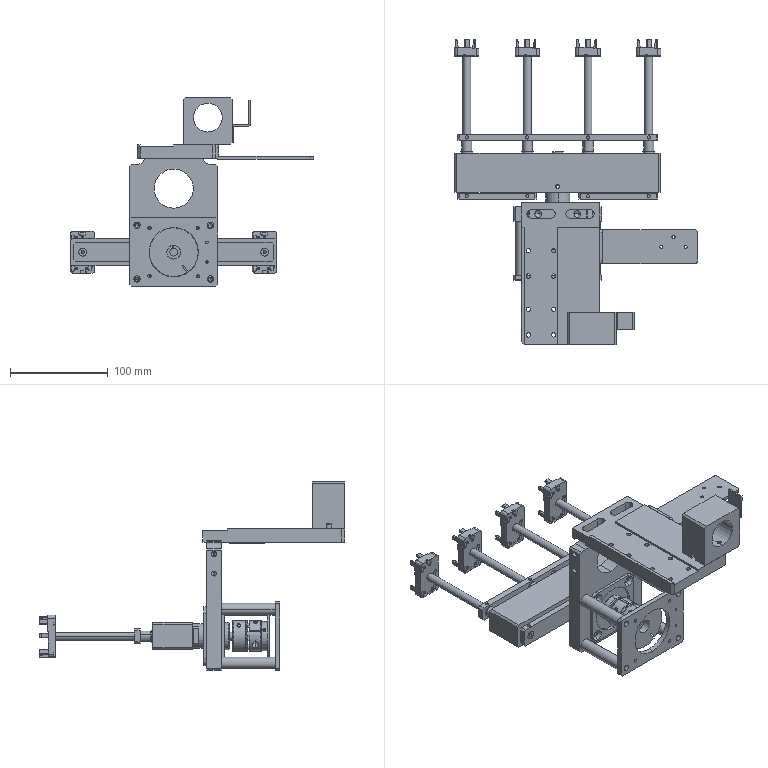Assembly | SolidWorks | mm | 68 component files | 68 solids | 1794 faces | box 248.4 x 312.2 x 193 mm | volume 766712 mm3 | plane 738 | cylinder 730 | cone 220 | spline 94 | torus 12 | commonest cylinder face diameters 2.5 x88 3.3 x72 8 x53 6 x53 4 x50 4.2 x48 4.5 x48 10 x36
Bill of materials:
H2020022-0402-1 | 4 | 45#Steel | Long, slender cylindrical rod or tube with a short, smaller-diameter stepped spigot at one end and an axial bore open at the other end.
H2020022-0446-1(3920) | 24 | 45#Steel | Elongated rectangular block with a sloped/tapered top surface toward one end, a small rounded tip, and a longitudinal step (rabbet) along one top edge that stops short of one end.
H2020022-0447-1(3920) | 4 | 45#Steel | Rectangular plate with rounded corners, a central round through hole, several rectangular pockets/notches near the edges, multiple small conical (countersunk-looking) holes, and a raised step on part of one face.
LOC71-D8-L40-E40-G30-2 | 4 |  | Flanged cylindrical sleeve: a hollow tube with a larger-diameter collar at one end and a straight through bore.
H2020022-0405-1 | 4 | Stainless Steel304 | Plain flat annular ring (washer-like) with a rectangular cross-section.
H2020022-0445-1(3920) | 2 | 45#Steel | Rectangular bar with chamfered corners, two through holes across its thickness near each end, and two smaller cross holes drilled from one long edge into the larger holes.
H2020022-0448-1(3920) | 1 | 45#Steel | Long, slender rectangular bar with chamfered corners, five evenly spaced through holes along its length, and four small cross holes from one long edge, at least some of which meet the main holes.
H2020022-0449-1(3920) | 1 | 6061 Aluminum Alloy | Rectangular block/bar with five holes through one face (the center hole smaller than the other four), chamfered end corners, and one small cross hole from the top face into the center hole.
RoundWireSpringYNWL-D8.5-L30 | 4 |  | Thin-walled cylindrical sleeve with thin rim/lip features at both ends; the rims look partial or offset, which suggests a seam or split.
BearingCH-NTN6304ZZ | 1 |  | Thick annular disc (spacer- or washer-like) with a central through hole and small rounded edges.
DowelPin5X15L | 2 |  | Solid cylindrical pin with chamfers at both ends.
H2020022-0406-1 | 2 | SUS304 | Thin square plate with rounded corners, a large central circular opening, and four corner through holes.
H2020022-0408-1 | 1 | Stainless Steel304 | Flat circular ring (washer-like annular disc) with a concentric central through-hole.
H2020022-0409-1 | 4 | 45#Steel | Long plain cylinder (tube or spacer-like) with a small concentric axial bore at the end.
H2020022-0411-1 | 1 | Stainless Steel304 | Thin rectangular plate with chamfered corners, a large central circular opening, four larger corner holes, and six smaller holes.
H2020022-0413-1 | 1 | 6061 Aluminum Alloy | Thick rectangular plate with two large circular through-openings of different sizes stacked along its length, several smaller through-holes, and a narrower top tab formed by rounded corner notches.
H2020022-0415-1 | 1 | 45#Steel | Stepped cylindrical shaft/hub: a larger-diameter collar between a medium-diameter end section and a smaller-diameter pin section; the pin has a cross-hole and a flat or notch.
H2020022-0418-1 | 1 | 6061 Aluminum Alloy | Rectangular machined plate with two elongated slots at one end, a grid of round through-holes, stepped/rabbeted edges, and small holes in one side face.
H2020022-0435-1 | 1 | 6061 Aluminum Alloy | Rectangular block with a large circular through-bore, chamfered edges along the bore direction, and small holes in one side face and inside the bore.
H2020022-0437-1 | 1 | 45#Steel | Thin circular flange disc with a central hole, a radial slit running from the outer edge, and a short cylindrical hub on one side that has radial cross-holes.
H2020022-0438-1 | 1 | 45#Steel | Knob- or flange-like disc with a chamfered rim, four equally spaced axial through-holes, and a solid cylindrical stub shaft centered on one face.
H2020022-0439-1 | 1 | Stainless Steel304 | Bent sheet-metal Z-shaped (offset) bracket: a tall flat flange, a horizontal web, and a short lower flange with two elongated slots.
H2020022-0443-1 | 1 | Stainless Steel304 | L-shaped bent bracket: a long flat base plate with three small holes near one end, and a short upturned flange with two larger holes.
YihadaCouplingDBA51-D32-d8-e14 | 1 |  | Cylindrical body with a central keyed bore, several transverse slits that make it look like a slit-type flexible shaft coupling, radial clamp holes, and modeled socket-head screws.
Mates:
1. concentric | H2020022-0413-1-1 face at (-30.964, 102.013, 280.197) dir (0, 1, 0) r 26 | H2020022-0415-1-1 face at (-30.964, 148.013, 280.197) dir (0, -1, 0) r 5
2. coincident | H2020022-0413-1-1 face at (-75.964, 102.013, 370.197) dir (0, -1, 0) | H2020022-0409-1-1 face at (-68.464, 102.013, 307.697) dir (0, 1, 0)
3. coincident | H2020022-0409-1-1 face at (-68.464, 47.013, 307.697) dir (0, -1, 0) | H2020022-0411-1-1 face at (-75.964, 47.013, 245.197) dir (0, 1, 0)
4. concentric | H2020022-0409-1-1 face at (-68.464, 47.013, 307.697) dir (0, -1, 0) r 2.1 | H2020022-0411-1-1 face at (-68.464, 42.013, 307.697) dir (0, -1, 0) r 3.25
5. coincident | H2020022-0409-1-2 face at (-68.464, 47.013, 252.697) dir (0, -1, 0) | H2020022-0411-1-1 face at (-75.964, 47.013, 245.197) dir (0, 1, 0)
6. coincident | H2020022-0409-1-4 face at (6.536, 47.013, 252.697) dir (0, -1, 0) | H2020022-0411-1-1 face at (-75.964, 47.013, 245.197) dir (0, 1, 0)
7. coincident | H2020022-0409-1-3 face at (6.536, 47.013, 307.697) dir (0, -1, 0) | H2020022-0411-1-1 face at (-75.964, 47.013, 245.197) dir (0, 1, 0)
8. concentric | H2020022-0409-1-3 face at (6.536, 47.013, 307.697) dir (0, -1, 0) r 2.1 | H2020022-0411-1-1 face at (6.536, 42.013, 307.697) dir (0, -1, 0) r 3.25
9. concentric | H2020022-0409-1-4 face at (6.536, 47.013, 252.697) dir (0, -1, 0) r 2.1 | H2020022-0411-1-1 face at (6.536, 42.013, 252.697) dir (0, -1, 0) r 3.25
10. concentric | H2020022-0409-1-2 face at (-68.464, 47.013, 252.697) dir (0, -1, 0) r 2.1 | H2020022-0411-1-1 face at (-68.464, 42.013, 252.697) dir (0, -1, 0) r 3.25
11. concentric | H2020022-0413-1-1 face at (6.536, 116.813, 252.697) dir (0, 1, 0) r 2.75 | H2020022-0409-1-4 face at (6.536, 102.013, 252.697) dir (0, 1, 0) r 2.1
12. concentric | H2020022-0413-1-1 face at (-30.964, 102.013, 280.197) dir (0, 1, 0) r 26 | BearingCH-NTN6304ZZ-1 face at (-30.964, 116.813, 280.197) dir (0, -1, 0) r 26
13. coincident | H2020022-0415-1-1 face at (-30.964, 116.813, 280.197) dir (0, -1, 0) | BearingCH-NTN6304ZZ-1 face at (-30.964, 116.813, 280.197) dir (0, 1, 0)
14. coincident | BearingCH-NTN6304ZZ-1 face at (-30.964, 101.813, 280.197) dir (0, -1, 0) | H2020022-0438-1-1 face at (-30.964, 101.813, 280.197) dir (0, 1, 0)
15. concentric | H2020022-0415-1-1 face at (-30.964, 116.813, 280.197) dir (0, -1, 0) r 10 | H2020022-0438-1-1 face at (-30.964, 81.813, 280.197) dir (0, 1, 0) r 4
16. coincident | 04LowerMaterialReceivingSwingAngleAssembly(3920)-1/H2020022-0449-1(3920)-2 face at (-135.964, 131.813, 294.197) dir (0, -1, 0) | H2020022-0415-1-1 face at (-30.964, 131.813, 280.197) dir (0, 1, 0)
17. concentric | 04LowerMaterialReceivingSwingAngleAssembly(3920)-1/H2020022-0449-1(3920)-2 face at (-30.964, 171.813, 280.197) dir (0, -1, 0) r 5 | H2020022-0415-1-1 face at (-30.964, 148.013, 280.197) dir (0, -1, 0) r 5
18. coincident | H2020022-0413-1-1 face at (-75.964, 116.813, 370.197) dir (0, 1, 0) | BearingCH-NTN6304ZZ-1 face at (-30.964, 116.813, 280.197) dir (0, 1, 0)
19. coincident | 04LowerMaterialReceivingSwingAngleAssembly(3920)-1/H2020022-0449-1(3920)-2 face at (-135.964, 171.813, 294.197) dir (0, 1, 0) | H2020022-0408-1-11 face at (-30.964, 171.813, 280.197) dir (0, -1, 0)
20. concentric | 04LowerMaterialReceivingSwingAngleAssembly(3920)-1/H2020022-0449-1(3920)-2 face at (-30.964, 171.813, 280.197) dir (0, -1, 0) r 5 | H2020022-0408-1-11 face at (-30.964, 173.313, 280.197) dir (0, -1, 0) r 2.05
21. coincident | H2020022-0435-1-1 face at (3.932, -24.187, 414.197) dir (0, -1, 0) | H2020022-0418-1-1 face at (-68.068, -24.187, 390.197) dir (0, -1, 0)
22. concentric | H2020022-0418-1-1 face at (-16.068, -7.687, 390.197) dir (0, 0, -1) r 2.5 | DowelPin5X15L-2 face at (-16.068, -7.687, 380.197) dir (0, 0, 1) r 2.5
23. coincident | H2020022-0435-1-1 face at (-21.068, -7.687, 395.197) dir (0, 0, -1) | DowelPin5X15L-2 face at (-16.068, -7.687, 395.197) dir (0, 0, 1)
24. concentric | H2020022-0418-1-1 face at (5.932, -7.687, 390.197) dir (0, 0, -1) r 2.5 | DowelPin5X15L-3 face at (5.932, -7.687, 395.197) dir (0, 0, -1) r 2.5
25. coincident | DowelPin5X15L-2 face at (-16.068, -7.687, 380.197) dir (0, 0, -1) | DowelPin5X15L-3 face at (5.932, -7.687, 380.197) dir (0, 0, -1)
26. parallel | 04LowerMaterialReceivingSwingAngleAssembly(3920)-1/H2020022-0449-1(3920)-2 face at (-135.964, 131.813, 266.197) dir (0, 0, -1) | H2020022-0413-1-1 face at (-75.964, 116.813, 245.197) dir (0, 0, -1)
27. concentric | H2020022-0415-1-1 face at (-30.964, 131.813, 280.197) dir (0, -1, 0) r 12.5 | H2020022-0406-1-1 face at (-30.964, 119.813, 280.197) dir (0, -1, 0) r 24
28. coincident | H2020022-0413-1-1 face at (-75.964, 116.813, 370.197) dir (0, 1, 0) | H2020022-0406-1-1 face at (-30.964, 116.813, 280.197) dir (0, -1, 0)
29. concentric | H2020022-0413-1-1 face at (-53.592, 116.813, 302.824) dir (0, 1, 0) r 2.1 | H2020022-0406-1-1 face at (-53.592, 119.813, 302.824) dir (0, 1, 0) r 2.75
30. concentric | H2020022-0438-1-1 face at (-30.964, 101.813, 280.197) dir (0, -1, 0) r 14 | H2020022-0406-1-2 face at (-30.964, 98.813, 280.197) dir (0, 1, 0) r 24
31. concentric | H2020022-0413-1-1 face at (-8.337, 116.813, 257.569) dir (0, 1, 0) r 2.1 | H2020022-0406-1-2 face at (-8.337, 98.813, 257.569) dir (0, -1, 0) r 2.75
32. concentric | H2020022-0438-1-1 face at (-30.964, 81.813, 280.197) dir (0, 1, 0) r 4 | YihadaCouplingDBA51-D32-d8-e14-1 face at (-30.964, 61.013, 280.197) dir (0, 1, 0) r 16
33. coincident | H2020022-0418-1-1 face at (11.932, 120.813, 390.197) dir (1, 0, 0) | H2020022-0443-1-1 face at (11.932, 93.313, 390.197) dir (-1, 0, 0)
34. concentric | H2020022-0418-1-1 face at (11.932, 85.813, 383.197) dir (1, 0, 0) r 1.65 | H2020022-0443-1-1 face at (11.932, 85.813, 383.197) dir (1, 0, 0) r 2.25
35. concentric | H2020022-0418-1-1 face at (11.932, 65.813, 383.197) dir (1, 0, 0) r 1.65 | H2020022-0443-1-1 face at (11.932, 65.813, 383.197) dir (1, 0, 0) r 2.25
36. coincident | H2020022-0435-1-1 face at (28.932, -24.187, 390.197) dir (1, 0, 0) | H2020022-0439-1-1 face at (28.932, 8.813, 392.658) dir (-1, 0, 0)
37. parallel | H2020022-0435-1-1 face at (3.932, 8.813, 414.197) dir (0, 1, 0) | H2020022-0439-1-1 face at (30.432, 8.813, 392.658) dir (0, 1, 0)
38. coincident | YihadaCouplingDBA51-D32-d8-e14-1 face at (-46.228, 61.013, 282.89) dir (0, -1, 0) | H2020022-0437-1-2 face at (-30.964, 61.013, 280.197) dir (0, 1, 0)
39. coincident | H2020022-0413-1-1 face at (-75.964, 116.813, 370.197) dir (0, 1, 0) | H2020022-0418-1-1 face at (11.932, 116.813, 378.197) dir (0, -1, 0)
40. coincident | H2020022-0413-1-1 face at (-0.9642, 116.813, 378.197) dir (0, 0, 1) | H2020022-0418-1-1 face at (-68.068, 120.813, 378.197) dir (0, 0, -1)
41. distance | H2020022-0437-1-2 face at (-30.964, 53.013, 280.197) dir (0, -1, 0) | H2020022-0411-1-1 face at (-75.964, 47.013, 245.197) dir (0, 1, 0)
42. slot | H2020022-0439-1-1 face at (47.432, -3.537, 401.158) dir (0, -1, 0) | H2020022-0435-1-1 face at (28.932, -5.187, 400.197) dir (1, 0, 0) r 1.25
43. coincident | BearingCH-NTN6304ZZ-1 face at (-30.964, 101.813, 280.197) dir (0, -1, 0) | H2020022-0406-1-2 face at (-30.964, 101.813, 280.197) dir (0, 1, 0)
44. concentric | 04LowerMaterialReceivingDieAssembly(3920)-3/H2020022-0402-1-1 face at (-133.5, 107.199, -14) dir (0, -1, 0) r 4 | H2020022-0448-1(3920)-3 face at (-133.5, 17.199, -14) dir (0, 1, 0) r 4
45. concentric | 04LowerMaterialReceivingDieAssembly(3920)-4/H2020022-0402-1-1 face at (52.5, 107.199, -14) dir (0, -1, 0) r 4 | H2020022-0448-1(3920)-3 face at (52.5, 17.199, -14) dir (0, 1, 0) r 4
46. distance | H2020022-0448-1(3920)-3 face at (-143, 17.199, -21.5) dir (0, -1, 0) | 04LowerMaterialReceivingDieAssembly(3920)-3/H2020022-0402-1-1 face at (-133.5, -42.801, -14) dir (0, -1, 0)
47. concentric | 04LowerMaterialReceivingDieAssembly(3920)-3/H2020022-0402-1-1 face at (-133.5, 107.199, -14) dir (0, -1, 0) r 4 | H2020022-0405-1-11 face at (-133.5, 5.699, -14) dir (0, -1, 0) r 4.1
48. coincident | H2020022-0405-1-11 face at (-133.5, 5.699, -14) dir (0, 1, 0) | H2020022-0405-1-10 face at (-9.5, 5.699, -14) dir (0, 1, 0)
49. coincident | H2020022-0405-1-11 face at (-133.5, 5.699, -14) dir (0, 1, 0) | H2020022-0405-1-9 face at (-71.5, 5.699, -14) dir (0, 1, 0)
50. concentric | 04LowerMaterialReceivingDieAssembly(3920)-2/H2020022-0402-1-1 face at (-71.5, 107.199, -14) dir (0, -1, 0) r 4 | H2020022-0405-1-9 face at (-71.5, 5.699, -14) dir (0, -1, 0) r 6
51. concentric | 04LowerMaterialReceivingDieAssembly(3920)-1/H2020022-0402-1-1 face at (-9.5, 107.199, -14) dir (0, -1, 0) r 4 | H2020022-0405-1-10 face at (-9.5, 5.699, -14) dir (0, -1, 0) r 6
52. coincident | H2020022-0405-1-11 face at (-133.5, 5.699, -14) dir (0, 1, 0) | H2020022-0405-1-8 face at (52.5, 5.699, -14) dir (0, 1, 0)
53. concentric | 04LowerMaterialReceivingDieAssembly(3920)-4/H2020022-0402-1-1 face at (52.5, 107.199, -14) dir (0, -1, 0) r 4 | H2020022-0405-1-8 face at (52.5, 5.699, -14) dir (0, -1, 0) r 4.1
54. concentric | 04LowerMaterialReceivingDieAssembly(3920)-3/H2020022-0402-1-1 face at (-133.5, 107.199, -14) dir (0, -1, 0) r 4 | RoundWireSpringYNWL-D8.5-L30-5 face at (-133.5, 6.064, -14) dir (0, 1, 0) r 5.25
55. concentric | 04LowerMaterialReceivingDieAssembly(3920)-4/H2020022-0402-1-1 face at (52.5, 107.199, -14) dir (0, -1, 0) r 4 | RoundWireSpringYNWL-D8.5-L30-7 face at (52.5, 6.064, -14) dir (0, 1, 0) r 5.25
56. concentric | 04LowerMaterialReceivingDieAssembly(3920)-1/H2020022-0402-1-1 face at (-9.5, 107.199, -14) dir (0, -1, 0) r 4 | RoundWireSpringYNWL-D8.5-L30-8 face at (-9.5, 6.064, -14) dir (0, 1, 0) r 5.25
57. concentric | 04LowerMaterialReceivingDieAssembly(3920)-2/H2020022-0402-1-1 face at (-71.5, 107.199, -14) dir (0, -1, 0) r 4 | RoundWireSpringYNWL-D8.5-L30-6 face at (-71.5, 6.064, -14) dir (0, 1, 0) r 5.25
58. coincident | H2020022-0449-1(3920)-2 face at (-145.5, -35.801, 0) dir (0, 0, 1) | 04LowerMaterialReceivingSwingAngleAssembly(3920) plane at (0, 0, 0) dir (0, 0, 1)
59. concentric | H2020022-0449-1(3920)-2 face at (-133.5, 0.1987, -14) dir (0, 1, 0) r 7.5 | EwellixBallBushingLOC71-D8-L40-E40-G30-7/LOC71-D8-L40-E40-G30-2-1 face at (-133.5, -495.801, -14) dir (0, 1, 0) r 6
60. coincident | H2020022-0449-1(3920)-2 face at (-145.5, 4.199, 0) dir (0, 1, 0) | EwellixBallBushingLOC71-D8-L40-E40-G30-7/LOC71-D8-L40-E40-G30-2-1 face at (-130.932, 4.199, -20.188) dir (0, 1, 0)
61. concentric | H2020022-0449-1(3920)-2 face at (-71.5, 0.1987, -14) dir (0, 1, 0) r 7.5 | EwellixBallBushingLOC71-D8-L40-E40-G30-4/LOC71-D8-L40-E40-G30-2-1 face at (-71.5, -495.801, -14) dir (0, 1, 0) r 6
62. coincident | H2020022-0449-1(3920)-2 face at (-145.5, 4.199, 0) dir (0, 1, 0) | EwellixBallBushingLOC71-D8-L40-E40-G30-4/LOC71-D8-L40-E40-G30-2-1 face at (-76.7, 4.199, -9.775) dir (0, 1, 0)
63. concentric | H2020022-0449-1(3920)-2 face at (-9.5, 0.1987, -14) dir (0, 1, 0) r 7.5 | EwellixBallBushingLOC71-D8-L40-E40-G30-5/LOC71-D8-L40-E40-G30-2-1 face at (-9.5, -495.801, -14) dir (0, 1, 0) r 6
64. coincident | H2020022-0449-1(3920)-2 face at (-145.5, 4.199, 0) dir (0, 1, 0) | EwellixBallBushingLOC71-D8-L40-E40-G30-5/LOC71-D8-L40-E40-G30-2-1 face at (-9.5, 4.199, -20.7) dir (0, 1, 0)
65. concentric | H2020022-0449-1(3920)-2 face at (52.5, 4.199, -14) dir (0, -1, 0) r 6 | EwellixBallBushingLOC71-D8-L40-E40-G30-6/LOC71-D8-L40-E40-G30-2-1 face at (52.5, -495.801, -14) dir (0, 1, 0) r 6
66. coincident | H2020022-0449-1(3920)-2 face at (-145.5, 4.199, 0) dir (0, 1, 0) | EwellixBallBushingLOC71-D8-L40-E40-G30-6/LOC71-D8-L40-E40-G30-2-1 face at (52.5, 4.199, -20.7) dir (0, 1, 0)
67. concentric | EwellixBallBushingLOC71-D8-L40-E40-G30-6/LOC71-D8-L40-E40-G30-2-1 face at (52.5, -495.801, -14) dir (0, 1, 0) r 6 | RoundWireSpringYNWL-D8.5-L30-7 face at (52.5, 6.064, -14) dir (0, 1, 0) r 5.25
68. coincident | EwellixBallBushingLOC71-D8-L40-E40-G30-6/LOC71-D8-L40-E40-G30-2-1 face at (52.5, 4.199, -20.7) dir (0, 1, 0) | H2020022-0405-1-8 face at (52.5, 4.199, -14) dir (0, -1, 0)
69. concentric | 04LowerMaterialReceivingDieAssembly(3920)-2/H2020022-0402-1-1 face at (-71.5, 107.199, -14) dir (0, -1, 0) r 4 | H2020022-0448-1(3920)-3 face at (-71.5, 17.199, -14) dir (0, 1, 0) r 4
70. concentric | EwellixBallBushingLOC71-D8-L40-E40-G30-5/LOC71-D8-L40-E40-G30-2-1 face at (-9.5, -495.801, -14) dir (0, 1, 0) r 5 | 04LowerMaterialReceivingDieAssembly(3920)-1/H2020022-0402-1-1 face at (-9.5, 107.199, -14) dir (0, -1, 0) r 4
71. distance | 04LowerMaterialReceivingDieAssembly(3920)-3/H2020022-0402-1-1 face at (-133.5, -42.801, -14) dir (0, -1, 0) | EwellixBallBushingLOC71-D8-L40-E40-G30-7/LOC71-D8-L40-E40-G30-2-1 face at (-131.584, -35.801, -18.618) dir (0, -1, 0)
72. parallel | 04LowerMaterialReceivingSwingAngleAssembly(3920) face at (-133.565, 112.524, -8) dir (0, 0, 1) | H2020022-0448-1(3920)-3 face at (-143, 23.199, -6.5) dir (0, 0, 1)
73. coincident | 04LowerMaterialReceivingSwingAngleAssembly(3920) face at (-71.565, 109.399, -7.287) dir (0, -1, 0) | 04LowerMaterialReceivingSwingAngleAssembly(3920) face at (-133.565, 109.399, -7.287) dir (0, -1, 0)
74. coincident | 04LowerMaterialReceivingSwingAngleAssembly(3920) face at (-9.565, 109.399, -7.287) dir (0, -1, 0) | 04LowerMaterialReceivingSwingAngleAssembly(3920) face at (-133.565, 109.399, -7.287) dir (0, -1, 0)
75. coincident | 04LowerMaterialReceivingSwingAngleAssembly(3920) face at (-133.565, 109.399, -7.287) dir (0, -1, 0) | 04LowerMaterialReceivingSwingAngleAssembly(3920) face at (52.435, 109.399, -7.287) dir (0, -1, 0)
76. concentric | H2020022-0449-1(3920)-2 face at (-133.5, 4.199, -14) dir (0, -1, 0) r 6 | 04LowerMaterialReceivingDieAssembly(3920)-3/H2020022-0402-1-1 face at (-133.5, 107.199, -14) dir (0, -1, 0) r 4
77. coincident | 04LowerMaterialReceivingSwingAngleAssembly(3920) face at (-71.565, 112.524, -8) dir (0, 0, 1) | 04LowerMaterialReceivingSwingAngleAssembly(3920) face at (-133.565, 112.524, -8) dir (0, 0, 1)
78. coincident | 04LowerMaterialReceivingSwingAngleAssembly(3920) face at (-9.565, 112.524, -8) dir (0, 0, 1) | 04LowerMaterialReceivingSwingAngleAssembly(3920) face at (-133.565, 112.524, -8) dir (0, 0, 1)
79. coincident | 04LowerMaterialReceivingSwingAngleAssembly(3920) face at (-133.565, 112.524, -8) dir (0, 0, 1) | 04LowerMaterialReceivingSwingAngleAssembly(3920) face at (52.435, 112.524, -8) dir (0, 0, 1)
80. coincident | 04LowerMaterialReceivingDieAssembly(3920)-1/H2020022-0447-1(3920)-1 face at (-9.5, 104.724, 7.5) dir (0, 0, 1) | 04LowerMaterialReceivingDieAssembly(3920)-4/H2020022-0447-1(3920)-1 face at (52.5, 104.724, 7.5) dir (0, 0, 1)
81. coincident | 04LowerMaterialReceivingDieAssembly(3920)-1/H2020022-0447-1(3920)-1 face at (-9.5, 104.724, 7.5) dir (0, 0, 1) | 04LowerMaterialReceivingDieAssembly(3920)-2/H2020022-0447-1(3920)-1 face at (-71.5, 104.724, 7.5) dir (0, 0, 1)
82. coincident | 04LowerMaterialReceivingDieAssembly(3920)-2/H2020022-0447-1(3920)-1 face at (-71.5, 104.724, 7.5) dir (0, 0, 1) | 04LowerMaterialReceivingDieAssembly(3920)-3/H2020022-0447-1(3920)-1 face at (-133.5, 104.724, 7.5) dir (0, 0, 1)
83. coincident | 04LowerMaterialReceivingDieAssembly(3920)-2/H2020022-0447-1(3920)-1 face at (-68.762, 112.399, -6.551) dir (0, 1, 0) | 04LowerMaterialReceivingDieAssembly(3920)-3/H2020022-0447-1(3920)-1 face at (-130.762, 112.399, -6.551) dir (0, 1, 0)
84. coincident | 04LowerMaterialReceivingDieAssembly(3920)-1/H2020022-0447-1(3920)-1 face at (-6.762, 112.399, -6.551) dir (0, 1, 0) | 04LowerMaterialReceivingDieAssembly(3920)-4/H2020022-0447-1(3920)-1 face at (55.238, 112.399, -6.551) dir (0, 1, 0)
85. coincident | 04LowerMaterialReceivingDieAssembly(3920)-1/H2020022-0447-1(3920)-1 face at (-6.762, 112.399, -6.551) dir (0, 1, 0) | 04LowerMaterialReceivingDieAssembly(3920)-2/H2020022-0447-1(3920)-1 face at (-68.762, 112.399, -6.551) dir (0, 1, 0)
86. concentric | 04LowerMaterialReceivingDieAssembly(3920)-3/H2020022-0402-1-1 face at (-133.5, 107.199, -14) dir (0, -1, 0) r 4 | H2020022-0445-1(3920)-3 face at (-133.5, -42.801, -14) dir (0, 1, 0) r 4
87. concentric | 04LowerMaterialReceivingDieAssembly(3920)-2/H2020022-0402-1-1 face at (-71.5, 107.199, -14) dir (0, -1, 0) r 4 | H2020022-0445-1(3920)-3 face at (-71.5, -42.801, -14) dir (0, 1, 0) r 4
88. concentric | 04LowerMaterialReceivingDieAssembly(3920)-1/H2020022-0402-1-1 face at (-9.5, 107.199, -14) dir (0, -1, 0) r 4 | H2020022-0445-1(3920)-4 face at (-9.5, -42.801, -14) dir (0, 1, 0) r 4
89. concentric | 04LowerMaterialReceivingDieAssembly(3920)-4/H2020022-0402-1-1 face at (52.5, 107.199, -14) dir (0, -1, 0) r 4 | H2020022-0445-1(3920)-4 face at (52.5, -42.801, -14) dir (0, 1, 0) r 4
90. coincident | 04LowerMaterialReceivingDieAssembly(3920)-3/H2020022-0402-1-1 face at (-133.5, -42.801, -14) dir (0, -1, 0) | H2020022-0445-1(3920)-3 face at (-143, -42.801, -24) dir (0, -1, 0)
91. coincident | 04LowerMaterialReceivingDieAssembly(3920)-1/H2020022-0402-1-1 face at (-9.5, -42.801, -14) dir (0, -1, 0) | H2020022-0445-1(3920)-4 face at (-19, -42.801, -24) dir (0, -1, 0)
92. coincident | H2020022-0402-1-1 face at (34.463, 205.724, 110.445) dir (0, 1, 0) | H2020022-0447-1(3920)-1 face at (24.538, 205.724, 133.249) dir (0, -1, 0)
93. coincident | H2020022-0402-1-1 face at (32.824, 199.4, 113.657) dir (-0.9933, 0, 0.1158) | H2020022-0447-1(3920)-1 face at (32.358, 202.724, 109.653) dir (0.9933, 0, -0.1158)
94. concentric | H2020022-0402-1-1 face at (34.463, 205.724, 110.445) dir (0, 1, 0) r 2.25 | H2020022-0447-1(3920)-1 face at (34.463, 213.674, 110.445) dir (0, 1, 0) r 3.25
95. coincident | H2020022-0447-1(3920)-1 face at (24.538, 205.724, 133.249) dir (0, -1, 0) | H2020022-0446-1(3920)-1 face at (43.378, 205.724, 112.621) dir (0, -1, 0)
96. coincident | H2020022-0447-1(3920)-1 face at (40.092, 389.208, 84.442) dir (-0.9933, 0, 0.1158) | H2020022-0446-1(3920)-1 face at (43.378, 222.724, 112.621) dir (0.9933, 0, -0.1158)
97. coincident | H2020022-0447-1(3920)-1 face at (40.389, 213.674, 112.969) dir (-0.1158, 0, -0.9933) | H2020022-0446-1(3920)-1 face at (43.378, 222.724, 112.621) dir (0.1158, 0, 0.9933)
98. coincident | H2020022-0447-1(3920)-1 face at (39.235, 214.724, 129.735) dir (-0.1158, 0, -0.9933) | H2020022-0446-1(3920)-2 face at (34.269, 222.724, 130.314) dir (0.1158, 0, 0.9933)
99. coincident | H2020022-0447-1(3920)-1 face at (38.886, 214.724, 126.745) dir (-0.9933, 0, 0.1158) | H2020022-0446-1(3920)-2 face at (39.235, 222.724, 129.735) dir (0.9933, 0, -0.1158)
100. coincident | H2020022-0447-1(3920)-1 face at (25.183, 214.724, 128.648) dir (0.9933, 0, -0.1158) | H2020022-0446-1(3920)-3 face at (24.604, 222.724, 123.682) dir (-0.9933, 0, 0.1158)
101. coincident | H2020022-0447-1(3920)-1 face at (28.173, 214.724, 128.299) dir (-0.1158, 0, -0.9933) | H2020022-0446-1(3920)-3 face at (25.183, 222.724, 128.648) dir (0.1158, 0, 0.9933)
102. coincident | H2020022-0447-1(3920)-1 face at (24.538, 205.724, 133.249) dir (0, -1, 0) | H2020022-0446-1(3920)-3 face at (24.604, 205.724, 123.682) dir (0, -1, 0)
103. coincident | H2020022-0447-1(3920)-1 face at (24.538, 205.724, 133.249) dir (0, -1, 0) | H2020022-0446-1(3920)-2 face at (34.269, 205.724, 130.314) dir (0, -1, 0)
104. coincident | H2020022-0447-1(3920)-1 face at (40.092, 389.208, 84.442) dir (-0.9933, 0, 0.1158) | H2020022-0446-1(3920)-5 face at (41.408, 222.724, 95.725) dir (0.9933, 0, -0.1158)
105. coincident | H2020022-0447-1(3920)-1 face at (40.437, 217.674, 90.805) dir (0.1158, 0, 0.9933) | H2020022-0446-1(3920)-5 face at (40.829, 222.724, 90.759) dir (-0.1158, 0, -0.9933)
106. coincident | H2020022-0447-1(3920)-1 face at (24.538, 205.724, 133.249) dir (0, -1, 0) | H2020022-0446-1(3920)-5 face at (41.408, 205.724, 95.725) dir (0, -1, 0)
107. coincident | H2020022-0447-1(3920)-1 face at (20.297, 389.208, 86.751) dir (0.9933, 0, -0.1158) | H2020022-0446-1(3920)-4 face at (21.034, 222.724, 93.068) dir (-0.9933, 0, 0.1158)
108. coincident | H2020022-0447-1(3920)-1 face at (21.034, 202.724, 93.068) dir (0.1158, 0, 0.9933) | H2020022-0446-1(3920)-4 face at (21.034, 222.724, 93.068) dir (-0.1158, 0, -0.9933)
109. coincident | H2020022-0447-1(3920)-1 face at (24.538, 205.724, 133.249) dir (0, -1, 0) | H2020022-0446-1(3920)-4 face at (21.034, 205.724, 93.068) dir (0, -1, 0)
110. coincident | H2020022-0447-1(3920)-1 face at (24.579, 205.674, 93.164) dir (-0.1158, 0, -0.9933) | H2020022-0446-1(3920)-6 face at (34.83, 222.724, 91.968) dir (0.1158, 0, 0.9933)
111. coincident | H2020022-0447-1(3920)-1 face at (34.806, 217.674, 91.758) dir (-0.9933, 0, 0.1158) | H2020022-0446-1(3920)-6 face at (34.483, 222.724, 88.988) dir (0.9933, 0, -0.1158)
112. coincident | H2020022-0447-1(3920)-1 face at (24.538, 205.724, 133.249) dir (0, -1, 0) | H2020022-0446-1(3920)-6 face at (34.483, 205.724, 88.988) dir (0, -1, 0)